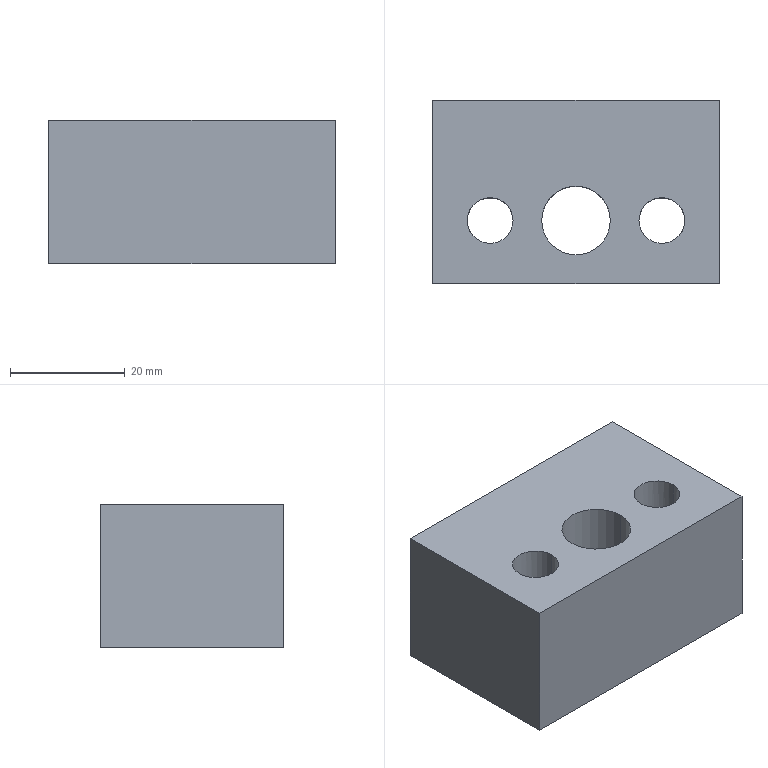Component | SolidWorks | BevelGearPlate2-2 | 1 solid | 18 faces | box 50 x 32 x 25 mm | volume 33376 mm3 | cylinder 10 | plane 6 | cone 2 | commonest cylinder face diameters 6.8 x4 8 x4 12 x2
build123d program:
from build123d import *

# Parameters (mm, degrees)
SKETCH1_W             = 50
SKETCH1_H             = 32
SKETCH1_R             = 4
SKETCH1_R_2           = 6
EXTRUDE1_DEPTH        = 25
M8_TAPPED_HOLE5_D     = 6.8
M8_TAPPED_HOLE5_DEPTH = 22.25
M8_TAPPED_HOLE5_TIP   = 2.043


with BuildPart() as part:
    # Sketch1 → Extrude1 (new body)
    with BuildSketch(Plane.XY):
        Rectangle(SKETCH1_W, SKETCH1_H)
        with Locations((-15, -5)):
            Circle(SKETCH1_R, mode=Mode.SUBTRACT)
        with Locations((15, -5)):
            Circle(SKETCH1_R, mode=Mode.SUBTRACT)
        with Locations((0, -5)):
            Circle(SKETCH1_R_2, mode=Mode.SUBTRACT)
    extrude(amount=EXTRUDE1_DEPTH)

    # M8 Tapped Hole5
    with Locations(Plane(origin=(0, 16, 0), x_dir=(-1, 0, 0), z_dir=(0, 1, 0))):
        with Locations((16, 12.5), (-16, 12.5)):
            Hole(M8_TAPPED_HOLE5_D / 2, depth=M8_TAPPED_HOLE5_DEPTH)
            with Locations((0, 0, -(M8_TAPPED_HOLE5_DEPTH + M8_TAPPED_HOLE5_TIP / 2))):  # 118° drill point
                Cone(0, M8_TAPPED_HOLE5_D / 2, M8_TAPPED_HOLE5_TIP, mode=Mode.SUBTRACT)


solid = part.part

# Placed as in the assembly
solid = solid.moved(Location((-143.621, 596.983, -92.215), (0, 0, 0)))
STEP:
#1=CARTESIAN_POINT('',(-6.402,23.306,-3.201));
#2=VERTEX_POINT('',#1);
#3=CARTESIAN_POINT('',(-6.284,23.459,-3.272));
#4=VERTEX_POINT('',#3);
#5=CARTESIAN_POINT('',(-6.402,23.306,-3.201));
#6=CARTESIAN_POINT('',(-6.402,23.311,-3.201));
#7=CARTESIAN_POINT('',(-6.402,23.316,-3.202));
#8=CARTESIAN_POINT('',(-6.401,23.325,-3.203));
#9=CARTESIAN_POINT('',(-6.401,23.329,-3.204));
#10=CARTESIAN_POINT('',(-6.398,23.342,-3.208));
#11=CARTESIAN_POINT('',(-6.396,23.351,-3.212));
#12=CARTESIAN_POINT('',(-6.391,23.366,-3.22));
#13=CARTESIAN_POINT('',(-6.387,23.374,-3.224));
#14=CARTESIAN_POINT('',(-6.38,23.388,-3.233));
#15=CARTESIAN_POINT('',(-6.375,23.395,-3.237));
#16=CARTESIAN_POINT('',(-6.365,23.408,-3.245));
#17=CARTESIAN_POINT('',(-6.36,23.414,-3.249));
#18=CARTESIAN_POINT('',(-6.348,23.426,-3.257));
#19=CARTESIAN_POINT('',(-6.341,23.432,-3.26));
#20=CARTESIAN_POINT('',(-6.326,23.441,-3.266));
#21=CARTESIAN_POINT('',(-6.319,23.446,-3.268));
#22=CARTESIAN_POINT('',(-6.302,23.454,-3.271));
#23=CARTESIAN_POINT('',(-6.293,23.457,-3.272));
#24=CARTESIAN_POINT('',(-6.284,23.459,-3.272));
#25=B_SPLINE_CURVE_WITH_KNOTS('',3,(#5,#6,#7,#8,#9,#10,#11,#12,#13,#14,#15,#16,#17,#18,#19,#20,#21,#22,#23,#24),.UNSPECIFIED.,.F.,.F.,(4,2,2,2,2,2,2,2,2,4),(0.001321,0.001673,0.002025,0.002729,0.003434,0.004138,0.004842,0.005547,0.006251,0.006955),.UNSPECIFIED.);
#26=EDGE_CURVE('',#2,#4,#25,.T.);
#27=ORIENTED_EDGE('',*,*,#26,.T.);
#28=CARTESIAN_POINT('',(-6.284,24.133,-3.272));
#29=VERTEX_POINT('',#28);
#30=CARTESIAN_POINT('',(-6.284,24.133,-3.272));
#31=DIRECTION('',(0.,1.,0.));
#32=VECTOR('',#31,39.37);
#33=LINE('',#30,#32);
#34=EDGE_CURVE('',#4,#29,#33,.T.);
#35=ORIENTED_EDGE('',*,*,#34,.T.);
#36=CARTESIAN_POINT('',(-6.284,24.133,-3.005));
#37=VERTEX_POINT('',#36);
#38=CARTESIAN_POINT('',(-6.284,24.133,-3.138));
#39=DIRECTION('',(0.,1.,0.));
#40=DIRECTION('',(0.,0.,1.));
#41=AXIS2_PLACEMENT_3D('',#38,#39,#40);
#42=CIRCLE('',#41,0.1339);
#43=EDGE_CURVE('',#29,#37,#42,.T.);
#44=ORIENTED_EDGE('',*,*,#43,.T.);
#45=CARTESIAN_POINT('',(-6.284,23.459,-3.005));
#46=VERTEX_POINT('',#45);
#47=CARTESIAN_POINT('',(-6.284,24.133,-3.005));
#48=DIRECTION('',(0.,1.,0.));
#49=VECTOR('',#48,39.37);
#50=LINE('',#47,#49);
#51=EDGE_CURVE('',#46,#37,#50,.T.);
#52=ORIENTED_EDGE('',*,*,#51,.F.);
#53=CARTESIAN_POINT('',(-6.402,23.306,-3.075));
#54=VERTEX_POINT('',#53);
#55=CARTESIAN_POINT('',(-6.284,23.459,-3.005));
#56=CARTESIAN_POINT('',(-6.293,23.457,-3.005));
#57=CARTESIAN_POINT('',(-6.302,23.453,-3.005));
#58=CARTESIAN_POINT('',(-6.319,23.446,-3.009));
#59=CARTESIAN_POINT('',(-6.326,23.441,-3.011));
#60=CARTESIAN_POINT('',(-6.341,23.432,-3.017));
#61=CARTESIAN_POINT('',(-6.348,23.426,-3.02));
#62=CARTESIAN_POINT('',(-6.36,23.414,-3.028));
#63=CARTESIAN_POINT('',(-6.365,23.408,-3.032));
#64=CARTESIAN_POINT('',(-6.375,23.395,-3.04));
#65=CARTESIAN_POINT('',(-6.38,23.388,-3.044));
#66=CARTESIAN_POINT('',(-6.387,23.374,-3.053));
#67=CARTESIAN_POINT('',(-6.391,23.366,-3.057));
#68=CARTESIAN_POINT('',(-6.396,23.351,-3.065));
#69=CARTESIAN_POINT('',(-6.398,23.342,-3.069));
#70=CARTESIAN_POINT('',(-6.402,23.325,-3.074));
#71=CARTESIAN_POINT('',(-6.402,23.316,-3.075));
#72=CARTESIAN_POINT('',(-6.402,23.306,-3.075));
#73=B_SPLINE_CURVE_WITH_KNOTS('',3,(#55,#56,#57,#58,#59,#60,#61,#62,#63,#64,#65,#66,#67,#68,#69,#70,#71,#72),.UNSPECIFIED.,.F.,.F.,(4,2,2,2,2,2,2,2,4),(0.01782,0.01853,0.01923,0.01993,0.02064,0.02134,0.02204,0.02274,0.02345),.UNSPECIFIED.);
#74=EDGE_CURVE('',#46,#54,#73,.T.);
#75=ORIENTED_EDGE('',*,*,#74,.T.);
#76=CARTESIAN_POINT('',(-6.395,23.257,-3.062));
#77=VERTEX_POINT('',#76);
#78=CARTESIAN_POINT('',(-6.402,23.306,-3.075));
#79=CARTESIAN_POINT('',(-6.402,23.298,-3.075));
#80=CARTESIAN_POINT('',(-6.402,23.289,-3.074));
#81=CARTESIAN_POINT('',(-6.399,23.273,-3.069));
#82=CARTESIAN_POINT('',(-6.397,23.265,-3.066));
#83=CARTESIAN_POINT('',(-6.395,23.257,-3.062));
#84=B_SPLINE_CURVE_WITH_KNOTS('',3,(#78,#79,#80,#81,#82,#83),.UNSPECIFIED.,.F.,.F.,(4,2,4),(0.02345,0.02411,0.02476),.UNSPECIFIED.);
#85=EDGE_CURVE('',#54,#77,#84,.T.);
#86=ORIENTED_EDGE('',*,*,#85,.T.);
#87=CARTESIAN_POINT('',(-6.395,23.257,-3.214));
#88=VERTEX_POINT('',#87);
#89=CARTESIAN_POINT('',(-6.284,23.257,-3.138));
#90=DIRECTION('',(0.,1.,0.));
#91=DIRECTION('',(0.,0.,1.));
#92=AXIS2_PLACEMENT_3D('',#89,#90,#91);
#93=CIRCLE('',#92,0.1339);
#94=EDGE_CURVE('',#88,#77,#93,.T.);
#95=ORIENTED_EDGE('',*,*,#94,.F.);
#96=CARTESIAN_POINT('',(-6.395,23.257,-3.214));
#97=CARTESIAN_POINT('',(-6.397,23.265,-3.211));
#98=CARTESIAN_POINT('',(-6.399,23.273,-3.208));
#99=CARTESIAN_POINT('',(-6.402,23.289,-3.203));
#100=CARTESIAN_POINT('',(-6.402,23.298,-3.201));
#101=CARTESIAN_POINT('',(-6.402,23.306,-3.201));
#102=B_SPLINE_CURVE_WITH_KNOTS('',3,(#96,#97,#98,#99,#100,#101),.UNSPECIFIED.,.F.,.F.,(4,2,4),(0.,0.0006604,0.001321),.UNSPECIFIED.);
#103=EDGE_CURVE('',#88,#2,#102,.T.);
#104=ORIENTED_EDGE('',*,*,#103,.T.);
#105=EDGE_LOOP('',(#27,#35,#44,#52,#75,#86,#95,#104));
#106=FACE_OUTER_BOUND('',#105,.T.);
#107=CARTESIAN_POINT('',(-6.284,24.133,-3.138));
#108=DIRECTION('',(0.,1.,0.));
#109=DIRECTION('',(0.,0.,1.));
#110=AXIS2_PLACEMENT_3D('',#107,#108,#109);
#111=CYLINDRICAL_SURFACE('',#110,0.1339);
#112=ADVANCED_FACE('',(#106),#111,.F.);
#113=CARTESIAN_POINT('',(-5.024,23.459,-3.005));
#114=VERTEX_POINT('',#113);
#115=CARTESIAN_POINT('',(-5.024,23.459,-3.272));
#116=VERTEX_POINT('',#115);
#117=CARTESIAN_POINT('',(-5.024,23.459,-3.005));
#118=CARTESIAN_POINT('',(-5.033,23.461,-3.005));
#119=CARTESIAN_POINT('',(-5.042,23.463,-3.005));
#120=CARTESIAN_POINT('',(-5.059,23.464,-3.009));
#121=CARTESIAN_POINT('',(-5.068,23.464,-3.012));
#122=CARTESIAN_POINT('',(-5.084,23.463,-3.018));
#123=CARTESIAN_POINT('',(-5.092,23.462,-3.023));
#124=CARTESIAN_POINT('',(-5.107,23.458,-3.033));
#125=CARTESIAN_POINT('',(-5.113,23.456,-3.038));
#126=CARTESIAN_POINT('',(-5.126,23.451,-3.05));
#127=CARTESIAN_POINT('',(-5.131,23.449,-3.057));
#128=CARTESIAN_POINT('',(-5.141,23.444,-3.071));
#129=CARTESIAN_POINT('',(-5.145,23.442,-3.079));
#130=CARTESIAN_POINT('',(-5.151,23.437,-3.095));
#131=CARTESIAN_POINT('',(-5.154,23.436,-3.103));
#132=CARTESIAN_POINT('',(-5.157,23.433,-3.121));
#133=CARTESIAN_POINT('',(-5.158,23.432,-3.13));
#134=CARTESIAN_POINT('',(-5.158,23.432,-3.147));
#135=CARTESIAN_POINT('',(-5.157,23.433,-3.156));
#136=CARTESIAN_POINT('',(-5.154,23.436,-3.174));
#137=CARTESIAN_POINT('',(-5.151,23.437,-3.182));
#138=CARTESIAN_POINT('',(-5.145,23.442,-3.198));
#139=CARTESIAN_POINT('',(-5.14,23.444,-3.206));
#140=CARTESIAN_POINT('',(-5.131,23.449,-3.22));
#141=CARTESIAN_POINT('',(-5.126,23.451,-3.227));
#142=CARTESIAN_POINT('',(-5.113,23.456,-3.239));
#143=CARTESIAN_POINT('',(-5.107,23.458,-3.244));
#144=CARTESIAN_POINT('',(-5.092,23.461,-3.254));
#145=CARTESIAN_POINT('',(-5.084,23.463,-3.258));
#146=CARTESIAN_POINT('',(-5.068,23.464,-3.265));
#147=CARTESIAN_POINT('',(-5.059,23.464,-3.268));
#148=CARTESIAN_POINT('',(-5.042,23.463,-3.271));
#149=CARTESIAN_POINT('',(-5.033,23.461,-3.272));
#150=CARTESIAN_POINT('',(-5.024,23.459,-3.272));
#151=B_SPLINE_CURVE_WITH_KNOTS('',3,(#117,#118,#119,#120,#121,#122,#123,#124,#125,#126,#127,#128,#129,#130,#131,#132,#133,#134,#135,#136,#137,#138,#139,#140,#141,#142,#143,#144,#145,#146,#147,#148,#149,#150),.UNSPECIFIED.,.F.,.F.,(4,2,2,2,2,2,2,2,2,2,2,2,2,2,2,2,4),(0.006955,0.007635,0.008314,0.008993,0.009673,0.01035,0.01103,0.01171,0.01239,0.01307,0.01375,0.01443,0.01511,0.01579,0.01647,0.01715,0.01782),.UNSPECIFIED.);
#152=EDGE_CURVE('',#114,#116,#151,.T.);
#153=ORIENTED_EDGE('',*,*,#152,.T.);
#154=CARTESIAN_POINT('',(-5.024,24.133,-3.272));
#155=VERTEX_POINT('',#154);
#156=CARTESIAN_POINT('',(-5.024,24.133,-3.272));
#157=DIRECTION('',(0.,1.,0.));
#158=VECTOR('',#157,39.37);
#159=LINE('',#156,#158);
#160=EDGE_CURVE('',#116,#155,#159,.T.);
#161=ORIENTED_EDGE('',*,*,#160,.T.);
#162=CARTESIAN_POINT('',(-5.024,24.133,-3.005));
#163=VERTEX_POINT('',#162);
#164=CARTESIAN_POINT('',(-5.024,24.133,-3.138));
#165=DIRECTION('',(0.,1.,0.));
#166=DIRECTION('',(0.,0.,1.));
#167=AXIS2_PLACEMENT_3D('',#164,#165,#166);
#168=CIRCLE('',#167,0.1339);
#169=EDGE_CURVE('',#155,#163,#168,.T.);
#170=ORIENTED_EDGE('',*,*,#169,.T.);
#171=CARTESIAN_POINT('',(-5.024,24.133,-3.005));
#172=DIRECTION('',(0.,1.,0.));
#173=VECTOR('',#172,39.37);
#174=LINE('',#171,#173);
#175=EDGE_CURVE('',#114,#163,#174,.T.);
#176=ORIENTED_EDGE('',*,*,#175,.F.);
#177=EDGE_LOOP('',(#153,#161,#170,#176));
#178=FACE_OUTER_BOUND('',#177,.T.);
#179=CARTESIAN_POINT('',(-5.024,24.133,-3.138));
#180=DIRECTION('',(0.,1.,0.));
#181=DIRECTION('',(0.,0.,1.));
#182=AXIS2_PLACEMENT_3D('',#179,#180,#181);
#183=CYLINDRICAL_SURFACE('',#182,0.1339);
#184=ADVANCED_FACE('',(#178),#183,.F.);
#185=CARTESIAN_POINT('',(-5.891,23.306,-2.646));
#186=VERTEX_POINT('',#185);
#187=CARTESIAN_POINT('',(-5.418,23.306,-2.646));
#188=VERTEX_POINT('',#187);
#189=CARTESIAN_POINT('',(-5.654,23.306,-2.646));
#190=DIRECTION('',(0.,0.,1.));
#191=DIRECTION('',(1.,0.,0.));
#192=AXIS2_PLACEMENT_3D('',#189,#190,#191);
#193=CIRCLE('',#192,0.2362);
#194=EDGE_CURVE('',#186,#188,#193,.T.);
#195=ORIENTED_EDGE('',*,*,#194,.T.);
#196=CARTESIAN_POINT('',(-5.418,23.306,-3.631));
#197=VERTEX_POINT('',#196);
#198=CARTESIAN_POINT('',(-5.418,23.306,-2.646));
#199=DIRECTION('',(0.,0.,-1.));
#200=VECTOR('',#199,39.37);
#201=LINE('',#198,#200);
#202=EDGE_CURVE('',#188,#197,#201,.T.);
#203=ORIENTED_EDGE('',*,*,#202,.T.);
#204=CARTESIAN_POINT('',(-5.891,23.306,-3.631));
#205=VERTEX_POINT('',#204);
#206=CARTESIAN_POINT('',(-5.654,23.306,-3.631));
#207=DIRECTION('',(0.,0.,1.));
#208=DIRECTION('',(1.,0.,0.));
#209=AXIS2_PLACEMENT_3D('',#206,#207,#208);
#210=CIRCLE('',#209,0.2362);
#211=EDGE_CURVE('',#205,#197,#210,.T.);
#212=ORIENTED_EDGE('',*,*,#211,.F.);
#213=CARTESIAN_POINT('',(-5.891,23.306,-2.646));
#214=DIRECTION('',(0.,0.,-1.));
#215=VECTOR('',#214,39.37);
#216=LINE('',#213,#215);
#217=EDGE_CURVE('',#186,#205,#216,.T.);
#218=ORIENTED_EDGE('',*,*,#217,.F.);
#219=EDGE_LOOP('',(#195,#203,#212,#218));
#220=FACE_OUTER_BOUND('',#219,.T.);
#221=CARTESIAN_POINT('',(-5.654,23.306,-2.646));
#222=DIRECTION('',(0.,0.,-1.));
#223=DIRECTION('',(-1.,0.,0.));
#224=AXIS2_PLACEMENT_3D('',#221,#222,#223);
#225=CYLINDRICAL_SURFACE('',#224,0.2362);
#226=ADVANCED_FACE('',(#220),#225,.F.);
#227=CARTESIAN_POINT('',(-5.221,23.306,-2.646));
#228=VERTEX_POINT('',#227);
#229=CARTESIAN_POINT('',(-4.906,23.306,-2.646));
#230=VERTEX_POINT('',#229);
#231=CARTESIAN_POINT('',(-5.064,23.306,-2.646));
#232=DIRECTION('',(0.,0.,1.));
#233=DIRECTION('',(1.,0.,0.));
#234=AXIS2_PLACEMENT_3D('',#231,#232,#233);
#235=CIRCLE('',#234,0.1575);
#236=EDGE_CURVE('',#228,#230,#235,.T.);
#237=ORIENTED_EDGE('',*,*,#236,.T.);
#238=CARTESIAN_POINT('',(-4.906,23.306,-3.075));
#239=VERTEX_POINT('',#238);
#240=CARTESIAN_POINT('',(-4.906,23.306,-2.646));
#241=DIRECTION('',(0.,0.,-1.));
#242=VECTOR('',#241,39.37);
#243=LINE('',#240,#242);
#244=EDGE_CURVE('',#230,#239,#243,.T.);
#245=ORIENTED_EDGE('',*,*,#244,.T.);
#246=CARTESIAN_POINT('',(-4.914,23.257,-3.062));
#247=VERTEX_POINT('',#246);
#248=CARTESIAN_POINT('',(-4.914,23.257,-3.062));
#249=CARTESIAN_POINT('',(-4.912,23.265,-3.066));
#250=CARTESIAN_POINT('',(-4.91,23.273,-3.069));
#251=CARTESIAN_POINT('',(-4.907,23.289,-3.074));
#252=CARTESIAN_POINT('',(-4.906,23.298,-3.075));
#253=CARTESIAN_POINT('',(-4.906,23.306,-3.075));
#254=B_SPLINE_CURVE_WITH_KNOTS('',3,(#248,#249,#250,#251,#252,#253),.UNSPECIFIED.,.F.,.F.,(4,2,4),(0.,0.0006604,0.001321),.UNSPECIFIED.);
#255=EDGE_CURVE('',#247,#239,#254,.T.);
#256=ORIENTED_EDGE('',*,*,#255,.F.);
#257=CARTESIAN_POINT('',(-4.914,23.257,-3.214));
#258=VERTEX_POINT('',#257);
#259=CARTESIAN_POINT('',(-4.914,23.257,-3.214));
#260=CARTESIAN_POINT('',(-4.916,23.252,-3.202));
#261=CARTESIAN_POINT('',(-4.918,23.248,-3.19));
#262=CARTESIAN_POINT('',(-4.921,23.241,-3.165));
#263=CARTESIAN_POINT('',(-4.922,23.238,-3.151));
#264=CARTESIAN_POINT('',(-4.922,23.239,-3.132));
#265=CARTESIAN_POINT('',(-4.921,23.239,-3.125));
#266=CARTESIAN_POINT('',(-4.921,23.241,-3.112));
#267=CARTESIAN_POINT('',(-4.92,23.243,-3.106));
#268=CARTESIAN_POINT('',(-4.918,23.248,-3.087));
#269=CARTESIAN_POINT('',(-4.916,23.252,-3.075));
#270=CARTESIAN_POINT('',(-4.914,23.257,-3.062));
#271=B_SPLINE_CURVE_WITH_KNOTS('',3,(#259,#260,#261,#262,#263,#264,#265,#266,#267,#268,#269,#270),.UNSPECIFIED.,.F.,.F.,(4,2,2,2,2,4),(0.0005242,0.001528,0.002532,0.003034,0.003536,0.004541),.UNSPECIFIED.);
#272=EDGE_CURVE('',#258,#247,#271,.T.);
#273=ORIENTED_EDGE('',*,*,#272,.F.);
#274=CARTESIAN_POINT('',(-4.906,23.306,-3.201));
#275=VERTEX_POINT('',#274);
#276=CARTESIAN_POINT('',(-4.906,23.306,-3.201));
#277=CARTESIAN_POINT('',(-4.906,23.298,-3.201));
#278=CARTESIAN_POINT('',(-4.907,23.289,-3.203));
#279=CARTESIAN_POINT('',(-4.91,23.273,-3.208));
#280=CARTESIAN_POINT('',(-4.912,23.265,-3.211));
#281=CARTESIAN_POINT('',(-4.914,23.257,-3.214));
#282=B_SPLINE_CURVE_WITH_KNOTS('',3,(#276,#277,#278,#279,#280,#281),.UNSPECIFIED.,.F.,.F.,(4,2,4),(0.02345,0.02411,0.02476),.UNSPECIFIED.);
#283=EDGE_CURVE('',#275,#258,#282,.T.);
#284=ORIENTED_EDGE('',*,*,#283,.F.);
#285=CARTESIAN_POINT('',(-4.906,23.306,-3.631));
#286=VERTEX_POINT('',#285);
#287=CARTESIAN_POINT('',(-4.906,23.306,-2.646));
#288=DIRECTION('',(0.,0.,-1.));
#289=VECTOR('',#288,39.37);
#290=LINE('',#287,#289);
#291=EDGE_CURVE('',#275,#286,#290,.T.);
#292=ORIENTED_EDGE('',*,*,#291,.T.);
#293=CARTESIAN_POINT('',(-5.221,23.306,-3.631));
#294=VERTEX_POINT('',#293);
#295=CARTESIAN_POINT('',(-5.064,23.306,-3.631));
#296=DIRECTION('',(0.,0.,1.));
#297=DIRECTION('',(1.,0.,0.));
#298=AXIS2_PLACEMENT_3D('',#295,#296,#297);
#299=CIRCLE('',#298,0.1575);
#300=EDGE_CURVE('',#294,#286,#299,.T.);
#301=ORIENTED_EDGE('',*,*,#300,.F.);
#302=CARTESIAN_POINT('',(-5.221,23.306,-2.646));
#303=DIRECTION('',(0.,0.,-1.));
#304=VECTOR('',#303,39.37);
#305=LINE('',#302,#304);
#306=EDGE_CURVE('',#228,#294,#305,.T.);
#307=ORIENTED_EDGE('',*,*,#306,.F.);
#308=EDGE_LOOP('',(#237,#245,#256,#273,#284,#292,#301,#307));
#309=FACE_OUTER_BOUND('',#308,.T.);
#310=CARTESIAN_POINT('',(-5.064,23.306,-2.646));
#311=DIRECTION('',(0.,0.,-1.));
#312=DIRECTION('',(-1.,0.,0.));
#313=AXIS2_PLACEMENT_3D('',#310,#311,#312);
#314=CYLINDRICAL_SURFACE('',#313,0.1575);
#315=ADVANCED_FACE('',(#309),#314,.F.);
#316=CARTESIAN_POINT('',(-6.402,23.306,-2.646));
#317=VERTEX_POINT('',#316);
#318=CARTESIAN_POINT('',(-6.087,23.306,-2.646));
#319=VERTEX_POINT('',#318);
#320=CARTESIAN_POINT('',(-6.245,23.306,-2.646));
#321=DIRECTION('',(0.,0.,1.));
#322=DIRECTION('',(1.,0.,0.));
#323=AXIS2_PLACEMENT_3D('',#320,#321,#322);
#324=CIRCLE('',#323,0.1575);
#325=EDGE_CURVE('',#317,#319,#324,.T.);
#326=ORIENTED_EDGE('',*,*,#325,.T.);
#327=CARTESIAN_POINT('',(-6.087,23.306,-3.631));
#328=VERTEX_POINT('',#327);
#329=CARTESIAN_POINT('',(-6.087,23.306,-2.646));
#330=DIRECTION('',(0.,0.,-1.));
#331=VECTOR('',#330,39.37);
#332=LINE('',#329,#331);
#333=EDGE_CURVE('',#319,#328,#332,.T.);
#334=ORIENTED_EDGE('',*,*,#333,.T.);
#335=CARTESIAN_POINT('',(-6.402,23.306,-3.631));
#336=VERTEX_POINT('',#335);
#337=CARTESIAN_POINT('',(-6.245,23.306,-3.631));
#338=DIRECTION('',(0.,0.,1.));
#339=DIRECTION('',(1.,0.,0.));
#340=AXIS2_PLACEMENT_3D('',#337,#338,#339);
#341=CIRCLE('',#340,0.1575);
#342=EDGE_CURVE('',#336,#328,#341,.T.);
#343=ORIENTED_EDGE('',*,*,#342,.F.);
#344=CARTESIAN_POINT('',(-6.402,23.306,-2.646));
#345=DIRECTION('',(0.,0.,-1.));
#346=VECTOR('',#345,39.37);
#347=LINE('',#344,#346);
#348=EDGE_CURVE('',#2,#336,#347,.T.);
#349=ORIENTED_EDGE('',*,*,#348,.F.);
#350=ORIENTED_EDGE('',*,*,#103,.F.);
#351=CARTESIAN_POINT('',(-6.395,23.257,-3.062));
#352=CARTESIAN_POINT('',(-6.393,23.252,-3.075));
#353=CARTESIAN_POINT('',(-6.391,23.248,-3.087));
#354=CARTESIAN_POINT('',(-6.388,23.241,-3.112));
#355=CARTESIAN_POINT('',(-6.387,23.238,-3.125));
#356=CARTESIAN_POINT('',(-6.387,23.239,-3.145));
#357=CARTESIAN_POINT('',(-6.387,23.239,-3.152));
#358=CARTESIAN_POINT('',(-6.388,23.241,-3.165));
#359=CARTESIAN_POINT('',(-6.389,23.243,-3.171));
#360=CARTESIAN_POINT('',(-6.391,23.248,-3.19));
#361=CARTESIAN_POINT('',(-6.393,23.252,-3.202));
#362=CARTESIAN_POINT('',(-6.395,23.257,-3.214));
#363=B_SPLINE_CURVE_WITH_KNOTS('',3,(#351,#352,#353,#354,#355,#356,#357,#358,#359,#360,#361,#362),.UNSPECIFIED.,.F.,.F.,(4,2,2,2,2,4),(0.0005242,0.001528,0.002532,0.003034,0.003536,0.004541),.UNSPECIFIED.);
#364=EDGE_CURVE('',#77,#88,#363,.T.);
#365=ORIENTED_EDGE('',*,*,#364,.F.);
#366=ORIENTED_EDGE('',*,*,#85,.F.);
#367=CARTESIAN_POINT('',(-6.402,23.306,-2.646));
#368=DIRECTION('',(0.,0.,-1.));
#369=VECTOR('',#368,39.37);
#370=LINE('',#367,#369);
#371=EDGE_CURVE('',#317,#54,#370,.T.);
#372=ORIENTED_EDGE('',*,*,#371,.F.);
#373=EDGE_LOOP('',(#326,#334,#343,#349,#350,#365,#366,#372));
#374=FACE_OUTER_BOUND('',#373,.T.);
#375=CARTESIAN_POINT('',(-6.245,23.306,-2.646));
#376=DIRECTION('',(0.,0.,-1.));
#377=DIRECTION('',(-1.,0.,0.));
#378=AXIS2_PLACEMENT_3D('',#375,#376,#377);
#379=CYLINDRICAL_SURFACE('',#378,0.1575);
#380=ADVANCED_FACE('',(#374),#379,.F.);
#381=ORIENTED_EDGE('',*,*,#236,.F.);
#382=CARTESIAN_POINT('',(-5.064,23.306,-2.646));
#383=DIRECTION('',(0.,0.,1.));
#384=DIRECTION('',(1.,0.,0.));
#385=AXIS2_PLACEMENT_3D('',#382,#383,#384);
#386=CIRCLE('',#385,0.1575);
#387=EDGE_CURVE('',#230,#228,#386,.T.);
#388=ORIENTED_EDGE('',*,*,#387,.F.);
#389=EDGE_LOOP('',(#381,#388));
#390=FACE_BOUND('',#389,.T.);
#391=CARTESIAN_POINT('',(-6.639,24.133,-2.646));
#392=VERTEX_POINT('',#391);
#393=CARTESIAN_POINT('',(-6.639,22.873,-2.646));
#394=VERTEX_POINT('',#393);
#395=CARTESIAN_POINT('',(-6.639,24.133,-2.646));
#396=DIRECTION('',(0.,-1.,0.));
#397=VECTOR('',#396,39.37);
#398=LINE('',#395,#397);
#399=EDGE_CURVE('',#392,#394,#398,.T.);
#400=ORIENTED_EDGE('',*,*,#399,.T.);
#401=CARTESIAN_POINT('',(-4.67,22.873,-2.646));
#402=VERTEX_POINT('',#401);
#403=CARTESIAN_POINT('',(-6.639,22.873,-2.646));
#404=DIRECTION('',(1.,0.,0.));
#405=VECTOR('',#404,39.37);
#406=LINE('',#403,#405);
#407=EDGE_CURVE('',#394,#402,#406,.T.);
#408=ORIENTED_EDGE('',*,*,#407,.T.);
#409=CARTESIAN_POINT('',(-4.67,24.133,-2.646));
#410=VERTEX_POINT('',#409);
#411=CARTESIAN_POINT('',(-4.67,24.133,-2.646));
#412=DIRECTION('',(0.,1.,0.));
#413=VECTOR('',#412,39.37);
#414=LINE('',#411,#413);
#415=EDGE_CURVE('',#402,#410,#414,.T.);
#416=ORIENTED_EDGE('',*,*,#415,.T.);
#417=CARTESIAN_POINT('',(-6.639,24.133,-2.646));
#418=DIRECTION('',(-1.,0.,0.));
#419=VECTOR('',#418,39.37);
#420=LINE('',#417,#419);
#421=EDGE_CURVE('',#410,#392,#420,.T.);
#422=ORIENTED_EDGE('',*,*,#421,.T.);
#423=EDGE_LOOP('',(#400,#408,#416,#422));
#424=FACE_OUTER_BOUND('',#423,.T.);
#425=ORIENTED_EDGE('',*,*,#325,.F.);
#426=CARTESIAN_POINT('',(-6.245,23.306,-2.646));
#427=DIRECTION('',(0.,0.,1.));
#428=DIRECTION('',(1.,0.,0.));
#429=AXIS2_PLACEMENT_3D('',#426,#427,#428);
#430=CIRCLE('',#429,0.1575);
#431=EDGE_CURVE('',#319,#317,#430,.T.);
#432=ORIENTED_EDGE('',*,*,#431,.F.);
#433=EDGE_LOOP('',(#425,#432));
#434=FACE_BOUND('',#433,.T.);
#435=ORIENTED_EDGE('',*,*,#194,.F.);
#436=CARTESIAN_POINT('',(-5.654,23.306,-2.646));
#437=DIRECTION('',(0.,0.,1.));
#438=DIRECTION('',(1.,0.,0.));
#439=AXIS2_PLACEMENT_3D('',#436,#437,#438);
#440=CIRCLE('',#439,0.2362);
#441=EDGE_CURVE('',#188,#186,#440,.T.);
#442=ORIENTED_EDGE('',*,*,#441,.F.);
#443=EDGE_LOOP('',(#435,#442));
#444=FACE_BOUND('',#443,.T.);
#445=CARTESIAN_POINT('',(-6.639,22.873,-2.646));
#446=DIRECTION('',(0.,0.,1.));
#447=DIRECTION('',(1.,0.,0.));
#448=AXIS2_PLACEMENT_3D('',#445,#446,#447);
#449=PLANE('',#448);
#450=ADVANCED_FACE('',(#390,#424,#434,#444),#449,.T.);
#451=CARTESIAN_POINT('',(-6.639,24.133,-3.631));
#452=VERTEX_POINT('',#451);
#453=CARTESIAN_POINT('',(-6.639,22.873,-3.631));
#454=VERTEX_POINT('',#453);
#455=CARTESIAN_POINT('',(-6.639,24.133,-3.631));
#456=DIRECTION('',(0.,-1.,0.));
#457=VECTOR('',#456,39.37);
#458=LINE('',#455,#457);
#459=EDGE_CURVE('',#452,#454,#458,.T.);
#460=ORIENTED_EDGE('',*,*,#459,.F.);
#461=CARTESIAN_POINT('',(-4.67,24.133,-3.631));
#462=VERTEX_POINT('',#461);
#463=CARTESIAN_POINT('',(-6.639,24.133,-3.631));
#464=DIRECTION('',(-1.,0.,0.));
#465=VECTOR('',#464,39.37);
#466=LINE('',#463,#465);
#467=EDGE_CURVE('',#462,#452,#466,.T.);
#468=ORIENTED_EDGE('',*,*,#467,.F.);
#469=CARTESIAN_POINT('',(-4.67,22.873,-3.631));
#470=VERTEX_POINT('',#469);
#471=CARTESIAN_POINT('',(-4.67,24.133,-3.631));
#472=DIRECTION('',(0.,1.,0.));
#473=VECTOR('',#472,39.37);
#474=LINE('',#471,#473);
#475=EDGE_CURVE('',#470,#462,#474,.T.);
#476=ORIENTED_EDGE('',*,*,#475,.F.);
#477=CARTESIAN_POINT('',(-6.639,22.873,-3.631));
#478=DIRECTION('',(1.,0.,0.));
#479=VECTOR('',#478,39.37);
#480=LINE('',#477,#479);
#481=EDGE_CURVE('',#454,#470,#480,.T.);
#482=ORIENTED_EDGE('',*,*,#481,.F.);
#483=EDGE_LOOP('',(#460,#468,#476,#482));
#484=FACE_OUTER_BOUND('',#483,.T.);
#485=ORIENTED_EDGE('',*,*,#342,.T.);
#486=CARTESIAN_POINT('',(-6.245,23.306,-3.631));
#487=DIRECTION('',(0.,0.,1.));
#488=DIRECTION('',(1.,0.,0.));
#489=AXIS2_PLACEMENT_3D('',#486,#487,#488);
#490=CIRCLE('',#489,0.1575);
#491=EDGE_CURVE('',#328,#336,#490,.T.);
#492=ORIENTED_EDGE('',*,*,#491,.T.);
#493=EDGE_LOOP('',(#485,#492));
#494=FACE_BOUND('',#493,.T.);
#495=ORIENTED_EDGE('',*,*,#300,.T.);
#496=CARTESIAN_POINT('',(-5.064,23.306,-3.631));
#497=DIRECTION('',(0.,0.,1.));
#498=DIRECTION('',(1.,0.,0.));
#499=AXIS2_PLACEMENT_3D('',#496,#497,#498);
#500=CIRCLE('',#499,0.1575);
#501=EDGE_CURVE('',#286,#294,#500,.T.);
#502=ORIENTED_EDGE('',*,*,#501,.T.);
#503=EDGE_LOOP('',(#495,#502));
#504=FACE_BOUND('',#503,.T.);
#505=ORIENTED_EDGE('',*,*,#211,.T.);
#506=CARTESIAN_POINT('',(-5.654,23.306,-3.631));
#507=DIRECTION('',(0.,0.,1.));
#508=DIRECTION('',(1.,0.,0.));
#509=AXIS2_PLACEMENT_3D('',#506,#507,#508);
#510=CIRCLE('',#509,0.2362);
#511=EDGE_CURVE('',#197,#205,#510,.T.);
#512=ORIENTED_EDGE('',*,*,#511,.T.);
#513=EDGE_LOOP('',(#505,#512));
#514=FACE_BOUND('',#513,.T.);
#515=CARTESIAN_POINT('',(-6.639,22.873,-3.631));
#516=DIRECTION('',(0.,0.,1.));
#517=DIRECTION('',(1.,0.,0.));
#518=AXIS2_PLACEMENT_3D('',#515,#516,#517);
#519=PLANE('',#518);
#520=ADVANCED_FACE('',(#484,#494,#504,#514),#519,.F.);
#521=ORIENTED_EDGE('',*,*,#459,.T.);
#522=CARTESIAN_POINT('',(-6.639,22.873,-2.646));
#523=DIRECTION('',(0.,0.,-1.));
#524=VECTOR('',#523,39.37);
#525=LINE('',#522,#524);
#526=EDGE_CURVE('',#394,#454,#525,.T.);
#527=ORIENTED_EDGE('',*,*,#526,.F.);
#528=ORIENTED_EDGE('',*,*,#399,.F.);
#529=CARTESIAN_POINT('',(-6.639,24.133,-2.646));
#530=DIRECTION('',(0.,0.,-1.));
#531=VECTOR('',#530,39.37);
#532=LINE('',#529,#531);
#533=EDGE_CURVE('',#392,#452,#532,.T.);
#534=ORIENTED_EDGE('',*,*,#533,.T.);
#535=EDGE_LOOP('',(#521,#527,#528,#534));
#536=FACE_OUTER_BOUND('',#535,.T.);
#537=CARTESIAN_POINT('',(-6.639,24.133,-2.646));
#538=DIRECTION('',(1.,0.,0.));
#539=DIRECTION('',(0.,0.,-1.));
#540=AXIS2_PLACEMENT_3D('',#537,#538,#539);
#541=PLANE('',#540);
#542=ADVANCED_FACE('',(#536),#541,.F.);
#543=ORIENTED_EDGE('',*,*,#481,.T.);
#544=CARTESIAN_POINT('',(-4.67,22.873,-2.646));
#545=DIRECTION('',(0.,0.,-1.));
#546=VECTOR('',#545,39.37);
#547=LINE('',#544,#546);
#548=EDGE_CURVE('',#402,#470,#547,.T.);
#549=ORIENTED_EDGE('',*,*,#548,.F.);
#550=ORIENTED_EDGE('',*,*,#407,.F.);
#551=ORIENTED_EDGE('',*,*,#526,.T.);
#552=EDGE_LOOP('',(#543,#549,#550,#551));
#553=FACE_OUTER_BOUND('',#552,.T.);
#554=CARTESIAN_POINT('',(-6.639,22.873,-2.646));
#555=DIRECTION('',(0.,1.,0.));
#556=DIRECTION('',(0.,0.,1.));
#557=AXIS2_PLACEMENT_3D('',#554,#555,#556);
#558=PLANE('',#557);
#559=ADVANCED_FACE('',(#553),#558,.F.);
#560=ORIENTED_EDGE('',*,*,#475,.T.);
#561=CARTESIAN_POINT('',(-4.67,24.133,-2.646));
#562=DIRECTION('',(0.,0.,-1.));
#563=VECTOR('',#562,39.37);
#564=LINE('',#561,#563);
#565=EDGE_CURVE('',#410,#462,#564,.T.);
#566=ORIENTED_EDGE('',*,*,#565,.F.);
#567=ORIENTED_EDGE('',*,*,#415,.F.);
#568=ORIENTED_EDGE('',*,*,#548,.T.);
#569=EDGE_LOOP('',(#560,#566,#567,#568));
#570=FACE_OUTER_BOUND('',#569,.T.);
#571=CARTESIAN_POINT('',(-4.67,24.133,-2.646));
#572=DIRECTION('',(-1.,0.,0.));
#573=DIRECTION('',(0.,0.,1.));
#574=AXIS2_PLACEMENT_3D('',#571,#572,#573);
#575=PLANE('',#574);
#576=ADVANCED_FACE('',(#570),#575,.F.);
#577=CARTESIAN_POINT('',(-6.284,24.133,-3.138));
#578=DIRECTION('',(0.,1.,0.));
#579=DIRECTION('',(0.,0.,1.));
#580=AXIS2_PLACEMENT_3D('',#577,#578,#579);
#581=CIRCLE('',#580,0.1339);
#582=EDGE_CURVE('',#37,#29,#581,.T.);
#583=ORIENTED_EDGE('',*,*,#582,.F.);
#584=ORIENTED_EDGE('',*,*,#43,.F.);
#585=EDGE_LOOP('',(#583,#584));
#586=FACE_BOUND('',#585,.T.);
#587=CARTESIAN_POINT('',(-5.024,24.133,-3.138));
#588=DIRECTION('',(0.,1.,0.));
#589=DIRECTION('',(0.,0.,1.));
#590=AXIS2_PLACEMENT_3D('',#587,#588,#589);
#591=CIRCLE('',#590,0.1339);
#592=EDGE_CURVE('',#163,#155,#591,.T.);
#593=ORIENTED_EDGE('',*,*,#592,.F.);
#594=ORIENTED_EDGE('',*,*,#169,.F.);
#595=EDGE_LOOP('',(#593,#594));
#596=FACE_BOUND('',#595,.T.);
#597=ORIENTED_EDGE('',*,*,#467,.T.);
#598=ORIENTED_EDGE('',*,*,#533,.F.);
#599=ORIENTED_EDGE('',*,*,#421,.F.);
#600=ORIENTED_EDGE('',*,*,#565,.T.);
#601=EDGE_LOOP('',(#597,#598,#599,#600));
#602=FACE_OUTER_BOUND('',#601,.T.);
#603=CARTESIAN_POINT('',(-6.639,24.133,-2.646));
#604=DIRECTION('',(0.,-1.,0.));
#605=DIRECTION('',(0.,0.,-1.));
#606=AXIS2_PLACEMENT_3D('',#603,#604,#605);
#607=PLANE('',#606);
#608=ADVANCED_FACE('',(#586,#596,#602),#607,.F.);
#609=ORIENTED_EDGE('',*,*,#333,.F.);
#610=ORIENTED_EDGE('',*,*,#431,.T.);
#611=ORIENTED_EDGE('',*,*,#371,.T.);
#612=ORIENTED_EDGE('',*,*,#74,.F.);
#613=CARTESIAN_POINT('',(-6.284,23.459,-3.272));
#614=CARTESIAN_POINT('',(-6.276,23.461,-3.272));
#615=CARTESIAN_POINT('',(-6.267,23.463,-3.271));
#616=CARTESIAN_POINT('',(-6.249,23.464,-3.268));
#617=CARTESIAN_POINT('',(-6.241,23.464,-3.265));
#618=CARTESIAN_POINT('',(-6.224,23.463,-3.258));
#619=CARTESIAN_POINT('',(-6.217,23.462,-3.254));
#620=CARTESIAN_POINT('',(-6.202,23.458,-3.244));
#621=CARTESIAN_POINT('',(-6.195,23.456,-3.239));
#622=CARTESIAN_POINT('',(-6.183,23.451,-3.226));
#623=CARTESIAN_POINT('',(-6.178,23.449,-3.22));
#624=CARTESIAN_POINT('',(-6.168,23.444,-3.206));
#625=CARTESIAN_POINT('',(-6.164,23.442,-3.198));
#626=CARTESIAN_POINT('',(-6.157,23.437,-3.182));
#627=CARTESIAN_POINT('',(-6.155,23.436,-3.174));
#628=CARTESIAN_POINT('',(-6.151,23.433,-3.156));
#629=CARTESIAN_POINT('',(-6.15,23.432,-3.147));
#630=CARTESIAN_POINT('',(-6.15,23.432,-3.129));
#631=CARTESIAN_POINT('',(-6.151,23.433,-3.121));
#632=CARTESIAN_POINT('',(-6.155,23.436,-3.103));
#633=CARTESIAN_POINT('',(-6.157,23.437,-3.095));
#634=CARTESIAN_POINT('',(-6.164,23.442,-3.079));
#635=CARTESIAN_POINT('',(-6.168,23.444,-3.071));
#636=CARTESIAN_POINT('',(-6.178,23.449,-3.057));
#637=CARTESIAN_POINT('',(-6.183,23.451,-3.05));
#638=CARTESIAN_POINT('',(-6.195,23.456,-3.038));
#639=CARTESIAN_POINT('',(-6.202,23.458,-3.032));
#640=CARTESIAN_POINT('',(-6.216,23.461,-3.023));
#641=CARTESIAN_POINT('',(-6.224,23.463,-3.018));
#642=CARTESIAN_POINT('',(-6.241,23.464,-3.012));
#643=CARTESIAN_POINT('',(-6.249,23.464,-3.009));
#644=CARTESIAN_POINT('',(-6.267,23.463,-3.005));
#645=CARTESIAN_POINT('',(-6.276,23.461,-3.005));
#646=CARTESIAN_POINT('',(-6.284,23.459,-3.005));
#647=B_SPLINE_CURVE_WITH_KNOTS('',3,(#613,#614,#615,#616,#617,#618,#619,#620,#621,#622,#623,#624,#625,#626,#627,#628,#629,#630,#631,#632,#633,#634,#635,#636,#637,#638,#639,#640,#641,#642,#643,#644,#645,#646),.UNSPECIFIED.,.F.,.F.,(4,2,2,2,2,2,2,2,2,2,2,2,2,2,2,2,4),(0.006955,0.007635,0.008314,0.008993,0.009673,0.01035,0.01103,0.01171,0.01239,0.01307,0.01375,0.01443,0.01511,0.01579,0.01647,0.01715,0.01782),.UNSPECIFIED.);
#648=EDGE_CURVE('',#4,#46,#647,.T.);
#649=ORIENTED_EDGE('',*,*,#648,.F.);
#650=ORIENTED_EDGE('',*,*,#26,.F.);
#651=ORIENTED_EDGE('',*,*,#348,.T.);
#652=ORIENTED_EDGE('',*,*,#491,.F.);
#653=EDGE_LOOP('',(#609,#610,#611,#612,#649,#650,#651,#652));
#654=FACE_OUTER_BOUND('',#653,.T.);
#655=CARTESIAN_POINT('',(-6.245,23.306,-2.646));
#656=DIRECTION('',(0.,0.,-1.));
#657=DIRECTION('',(-1.,0.,0.));
#658=AXIS2_PLACEMENT_3D('',#655,#656,#657);
#659=CYLINDRICAL_SURFACE('',#658,0.1575);
#660=ADVANCED_FACE('',(#654),#659,.F.);
#661=ORIENTED_EDGE('',*,*,#244,.F.);
#662=ORIENTED_EDGE('',*,*,#387,.T.);
#663=ORIENTED_EDGE('',*,*,#306,.T.);
#664=ORIENTED_EDGE('',*,*,#501,.F.);
#665=ORIENTED_EDGE('',*,*,#291,.F.);
#666=CARTESIAN_POINT('',(-5.024,23.459,-3.272));
#667=CARTESIAN_POINT('',(-5.016,23.457,-3.272));
#668=CARTESIAN_POINT('',(-5.007,23.453,-3.271));
#669=CARTESIAN_POINT('',(-4.99,23.446,-3.268));
#670=CARTESIAN_POINT('',(-4.982,23.441,-3.266));
#671=CARTESIAN_POINT('',(-4.968,23.432,-3.26));
#672=CARTESIAN_POINT('',(-4.961,23.426,-3.257));
#673=CARTESIAN_POINT('',(-4.949,23.414,-3.249));
#674=CARTESIAN_POINT('',(-4.943,23.408,-3.245));
#675=CARTESIAN_POINT('',(-4.933,23.395,-3.237));
#676=CARTESIAN_POINT('',(-4.929,23.388,-3.232));
#677=CARTESIAN_POINT('',(-4.921,23.374,-3.224));
#678=CARTESIAN_POINT('',(-4.918,23.366,-3.22));
#679=CARTESIAN_POINT('',(-4.912,23.351,-3.212));
#680=CARTESIAN_POINT('',(-4.91,23.342,-3.208));
#681=CARTESIAN_POINT('',(-4.907,23.325,-3.203));
#682=CARTESIAN_POINT('',(-4.906,23.316,-3.201));
#683=CARTESIAN_POINT('',(-4.906,23.306,-3.201));
#684=B_SPLINE_CURVE_WITH_KNOTS('',3,(#666,#667,#668,#669,#670,#671,#672,#673,#674,#675,#676,#677,#678,#679,#680,#681,#682,#683),.UNSPECIFIED.,.F.,.F.,(4,2,2,2,2,2,2,2,4),(0.01782,0.01853,0.01923,0.01993,0.02064,0.02134,0.02204,0.02274,0.02345),.UNSPECIFIED.);
#685=EDGE_CURVE('',#116,#275,#684,.T.);
#686=ORIENTED_EDGE('',*,*,#685,.F.);
#687=ORIENTED_EDGE('',*,*,#152,.F.);
#688=CARTESIAN_POINT('',(-4.906,23.306,-3.075));
#689=CARTESIAN_POINT('',(-4.906,23.311,-3.075));
#690=CARTESIAN_POINT('',(-4.907,23.316,-3.075));
#691=CARTESIAN_POINT('',(-4.907,23.325,-3.074));
#692=CARTESIAN_POINT('',(-4.908,23.329,-3.072));
#693=CARTESIAN_POINT('',(-4.91,23.342,-3.068));
#694=CARTESIAN_POINT('',(-4.912,23.351,-3.065));
#695=CARTESIAN_POINT('',(-4.918,23.366,-3.057));
#696=CARTESIAN_POINT('',(-4.921,23.374,-3.053));
#697=CARTESIAN_POINT('',(-4.929,23.388,-3.044));
#698=CARTESIAN_POINT('',(-4.934,23.395,-3.04));
#699=CARTESIAN_POINT('',(-4.943,23.408,-3.032));
#700=CARTESIAN_POINT('',(-4.949,23.414,-3.028));
#701=CARTESIAN_POINT('',(-4.961,23.426,-3.02));
#702=CARTESIAN_POINT('',(-4.968,23.432,-3.017));
#703=CARTESIAN_POINT('',(-4.982,23.441,-3.011));
#704=CARTESIAN_POINT('',(-4.99,23.446,-3.009));
#705=CARTESIAN_POINT('',(-5.007,23.454,-3.005));
#706=CARTESIAN_POINT('',(-5.015,23.457,-3.005));
#707=CARTESIAN_POINT('',(-5.024,23.459,-3.005));
#708=B_SPLINE_CURVE_WITH_KNOTS('',3,(#688,#689,#690,#691,#692,#693,#694,#695,#696,#697,#698,#699,#700,#701,#702,#703,#704,#705,#706,#707),.UNSPECIFIED.,.F.,.F.,(4,2,2,2,2,2,2,2,2,4),(0.001321,0.001673,0.002025,0.002729,0.003434,0.004138,0.004842,0.005547,0.006251,0.006955),.UNSPECIFIED.);
#709=EDGE_CURVE('',#239,#114,#708,.T.);
#710=ORIENTED_EDGE('',*,*,#709,.F.);
#711=EDGE_LOOP('',(#661,#662,#663,#664,#665,#686,#687,#710));
#712=FACE_OUTER_BOUND('',#711,.T.);
#713=CARTESIAN_POINT('',(-5.064,23.306,-2.646));
#714=DIRECTION('',(0.,0.,-1.));
#715=DIRECTION('',(-1.,0.,0.));
#716=AXIS2_PLACEMENT_3D('',#713,#714,#715);
#717=CYLINDRICAL_SURFACE('',#716,0.1575);
#718=ADVANCED_FACE('',(#712),#717,.F.);
#719=ORIENTED_EDGE('',*,*,#202,.F.);
#720=ORIENTED_EDGE('',*,*,#441,.T.);
#721=ORIENTED_EDGE('',*,*,#217,.T.);
#722=ORIENTED_EDGE('',*,*,#511,.F.);
#723=EDGE_LOOP('',(#719,#720,#721,#722));
#724=FACE_OUTER_BOUND('',#723,.T.);
#725=CARTESIAN_POINT('',(-5.654,23.306,-2.646));
#726=DIRECTION('',(0.,0.,-1.));
#727=DIRECTION('',(-1.,0.,0.));
#728=AXIS2_PLACEMENT_3D('',#725,#726,#727);
#729=CYLINDRICAL_SURFACE('',#728,0.2362);
#730=ADVANCED_FACE('',(#724),#729,.F.);
#731=ORIENTED_EDGE('',*,*,#272,.T.);
#732=CARTESIAN_POINT('',(-5.024,23.257,-3.138));
#733=DIRECTION('',(0.,1.,0.));
#734=DIRECTION('',(0.,0.,1.));
#735=AXIS2_PLACEMENT_3D('',#732,#733,#734);
#736=CIRCLE('',#735,0.1339);
#737=EDGE_CURVE('',#247,#258,#736,.T.);
#738=ORIENTED_EDGE('',*,*,#737,.T.);
#739=EDGE_LOOP('',(#731,#738));
#740=FACE_OUTER_BOUND('',#739,.T.);
#741=CARTESIAN_POINT('',(-5.024,23.257,-3.138));
#742=DIRECTION('',(0.,1.,0.));
#743=DIRECTION('',(0.,0.,1.));
#744=AXIS2_PLACEMENT_3D('',#741,#742,#743);
#745=CONICAL_SURFACE('',#744,0.1339,1.03);
#746=ADVANCED_FACE('',(#740),#745,.F.);
#747=ORIENTED_EDGE('',*,*,#160,.F.);
#748=ORIENTED_EDGE('',*,*,#685,.T.);
#749=ORIENTED_EDGE('',*,*,#283,.T.);
#750=ORIENTED_EDGE('',*,*,#737,.F.);
#751=ORIENTED_EDGE('',*,*,#255,.T.);
#752=ORIENTED_EDGE('',*,*,#709,.T.);
#753=ORIENTED_EDGE('',*,*,#175,.T.);
#754=ORIENTED_EDGE('',*,*,#592,.T.);
#755=EDGE_LOOP('',(#747,#748,#749,#750,#751,#752,#753,#754));
#756=FACE_OUTER_BOUND('',#755,.T.);
#757=CARTESIAN_POINT('',(-5.024,24.133,-3.138));
#758=DIRECTION('',(0.,1.,0.));
#759=DIRECTION('',(0.,0.,1.));
#760=AXIS2_PLACEMENT_3D('',#757,#758,#759);
#761=CYLINDRICAL_SURFACE('',#760,0.1339);
#762=ADVANCED_FACE('',(#756),#761,.F.);
#763=ORIENTED_EDGE('',*,*,#364,.T.);
#764=ORIENTED_EDGE('',*,*,#94,.T.);
#765=EDGE_LOOP('',(#763,#764));
#766=FACE_OUTER_BOUND('',#765,.T.);
#767=CARTESIAN_POINT('',(-6.284,23.257,-3.138));
#768=DIRECTION('',(0.,1.,0.));
#769=DIRECTION('',(0.,0.,1.));
#770=AXIS2_PLACEMENT_3D('',#767,#768,#769);
#771=CONICAL_SURFACE('',#770,0.1339,1.03);
#772=ADVANCED_FACE('',(#766),#771,.F.);
#773=ORIENTED_EDGE('',*,*,#34,.F.);
#774=ORIENTED_EDGE('',*,*,#648,.T.);
#775=ORIENTED_EDGE('',*,*,#51,.T.);
#776=ORIENTED_EDGE('',*,*,#582,.T.);
#777=EDGE_LOOP('',(#773,#774,#775,#776));
#778=FACE_OUTER_BOUND('',#777,.T.);
#779=CARTESIAN_POINT('',(-6.284,24.133,-3.138));
#780=DIRECTION('',(0.,1.,0.));
#781=DIRECTION('',(0.,0.,1.));
#782=AXIS2_PLACEMENT_3D('',#779,#780,#781);
#783=CYLINDRICAL_SURFACE('',#782,0.1339);
#784=ADVANCED_FACE('',(#778),#783,.F.);
#785=CLOSED_SHELL('',(#112,#184,#226,#315,#380,#450,#520,#542,#559,#576,#608,#660,#718,#730,#746,#762,#772,#784));
#786=MANIFOLD_SOLID_BREP('',#785);
#787=CARTESIAN_POINT('',(0.,0.,0.));
#788=DIRECTION('',(0.,0.,1.));
#789=DIRECTION('',(1.,0.,0.));
#790=AXIS2_PLACEMENT_3D('',#787,#788,#789);
#791=(LENGTH_UNIT()NAMED_UNIT(*)SI_UNIT($,.METRE.));
#792=LENGTH_MEASURE_WITH_UNIT(LENGTH_MEASURE(0.0254),#791);
#793=DIMENSIONAL_EXPONENTS(1.,0.,0.,0.,0.,0.,0.);
#794=(CONVERSION_BASED_UNIT('',#792)LENGTH_UNIT()NAMED_UNIT(#793));
#795=UNCERTAINTY_MEASURE_WITH_UNIT(LENGTH_MEASURE(0.00001),#794,'','');
#796=(NAMED_UNIT(*)PLANE_ANGLE_UNIT()SI_UNIT($,.RADIAN.));
#797=(NAMED_UNIT(*)SI_UNIT($,.STERADIAN.)SOLID_ANGLE_UNIT());
#798=(GEOMETRIC_REPRESENTATION_CONTEXT(3)GLOBAL_UNCERTAINTY_ASSIGNED_CONTEXT((#795))GLOBAL_UNIT_ASSIGNED_CONTEXT((#794,#796,#797))REPRESENTATION_CONTEXT('',''));
#799=ADVANCED_BREP_SHAPE_REPRESENTATION('',(#786,#790),#798);
#800=COLOUR_RGB('',0.7922,0.8196,0.9333);
#801=FILL_AREA_STYLE_COLOUR('',#800);
#802=FILL_AREA_STYLE('',(#801));
#803=SURFACE_STYLE_FILL_AREA(#802);
#804=SURFACE_SIDE_STYLE('',(#803));
#805=SURFACE_STYLE_USAGE(.BOTH.,#804);
#806=PRESENTATION_STYLE_ASSIGNMENT((#805));
#807=STYLED_ITEM('',(#806),#786);
#808=PRESENTATION_LAYER_ASSIGNMENT('','',(#807));
#809=(LENGTH_UNIT()NAMED_UNIT(*)SI_UNIT($,.METRE.));
#810=LENGTH_MEASURE_WITH_UNIT(LENGTH_MEASURE(0.0254),#809);
#811=DIMENSIONAL_EXPONENTS(1.,0.,0.,0.,0.,0.,0.);
#812=(CONVERSION_BASED_UNIT('',#810)LENGTH_UNIT()NAMED_UNIT(#811));
#813=UNCERTAINTY_MEASURE_WITH_UNIT(LENGTH_MEASURE(0.00001),#812,'','');
#814=(NAMED_UNIT(*)PLANE_ANGLE_UNIT()SI_UNIT($,.RADIAN.));
#815=(NAMED_UNIT(*)SI_UNIT($,.STERADIAN.)SOLID_ANGLE_UNIT());
#816=(GEOMETRIC_REPRESENTATION_CONTEXT(3)GLOBAL_UNCERTAINTY_ASSIGNED_CONTEXT((#813))GLOBAL_UNIT_ASSIGNED_CONTEXT((#812,#814,#815))REPRESENTATION_CONTEXT('',''));
#817=MECHANICAL_DESIGN_GEOMETRIC_PRESENTATION_REPRESENTATION('',(#807),#816);